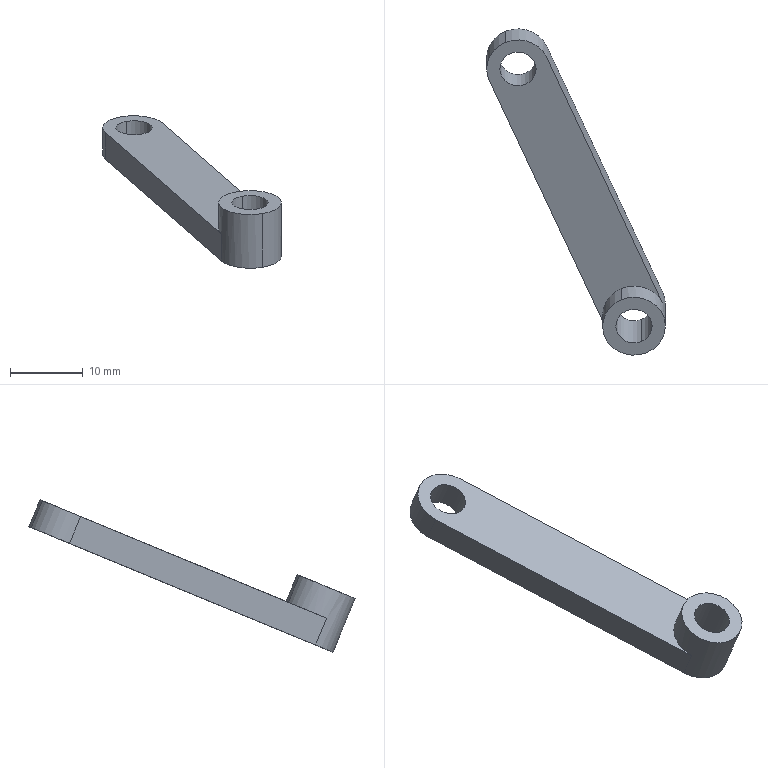Component | SolidWorks | ConnectingRod-B-1 | 1 solid | 13 faces | box 24.62 x 44.93 x 21 mm | volume 1615 mm3 | cylinder 8 | plane 5 | commonest cylinder face diameters 5 x4 8.636 x4
build123d program:
from build123d import *

# Parameters (mm, degrees)
SKETCH1_R           = 2.5
BOSS_EXTRUDE1_DEPTH = 2
SKETCH2_R           = 4.318
SKETCH2_R_2         = 2.5
BOSS_EXTRUDE2_DEPTH = 4


with BuildPart() as part:
    # Sketch1 → Boss-Extrude1 (new, symmetric)
    with BuildSketch(Plane.XY):
        with BuildLine():
            Line((0, 4.318), (40, 4.318))
            ThreePointArc((40, 4.318), (44.318, 0), (40, -4.318))
            Line((40, -4.318), (0, -4.318))
            ThreePointArc((0, -4.318), (-4.318, 0), (0, 4.318))
        make_face()
        Circle(SKETCH1_R, mode=Mode.SUBTRACT)
        with Locations((40, 0)):
            Circle(SKETCH1_R, mode=Mode.SUBTRACT)
    extrude(amount=BOSS_EXTRUDE1_DEPTH, both=True)

    # Sketch2 → Boss-Extrude2 (add)
    with BuildSketch(Plane.XY.offset(2)):
        with Locations(Location((40, 0, 0), (0, 0, 90))):
            Circle(SKETCH2_R)
        with Locations((40, 0)):
            Circle(SKETCH2_R_2, mode=Mode.SUBTRACT)
    extrude(amount=BOSS_EXTRUDE2_DEPTH)


solid = part.part

# Placed as in the assembly
solid = solid.moved(Location((321.124, 13.827, -7.578), (22.448, 0, -66.452)))
STEP:
#1=COLOUR_RGB('',0.7922,0.8196,0.9333);
#2=FILL_AREA_STYLE_COLOUR('',#1);
#3=FILL_AREA_STYLE('',(#2));
#4=SURFACE_STYLE_FILL_AREA(#3);
#5=SURFACE_SIDE_STYLE('',(#4));
#6=SURFACE_STYLE_USAGE(.BOTH.,#5);
#7=PRESENTATION_STYLE_ASSIGNMENT((#6));
#8=CARTESIAN_POINT('',(13.233,-0.7967,-0.5968));
#9=VERTEX_POINT('',#8);
#10=CARTESIAN_POINT('',(13.311,-0.9635,-0.6657));
#11=VERTEX_POINT('',#10);
#12=CARTESIAN_POINT('',(13.272,-0.8801,-0.6313));
#13=DIRECTION('',(0.,-0.3818,0.9242));
#14=DIRECTION('',(0.3995,-0.8473,-0.3501));
#15=AXIS2_PLACEMENT_3D('',#12,#13,#14);
#16=CIRCLE('',#15,0.09843);
#17=EDGE_CURVE('',#9,#11,#16,.T.);
#18=ORIENTED_EDGE('',*,*,#17,.T.);
#19=CARTESIAN_POINT('',(13.311,-0.8432,-0.9568));
#20=VERTEX_POINT('',#19);
#21=CARTESIAN_POINT('',(13.311,-0.9034,-0.8113));
#22=DIRECTION('',(-0.,0.3818,-0.9242));
#23=VECTOR('',#22,39.37);
#24=LINE('',#21,#23);
#25=EDGE_CURVE('',#11,#20,#24,.T.);
#26=ORIENTED_EDGE('',*,*,#25,.T.);
#27=CARTESIAN_POINT('',(13.233,-0.6764,-0.8879));
#28=VERTEX_POINT('',#27);
#29=CARTESIAN_POINT('',(13.272,-0.7598,-0.9224));
#30=DIRECTION('',(0.,-0.3818,0.9242));
#31=DIRECTION('',(0.3995,-0.8473,-0.3501));
#32=AXIS2_PLACEMENT_3D('',#29,#30,#31);
#33=CIRCLE('',#32,0.09843);
#34=EDGE_CURVE('',#28,#20,#33,.T.);
#35=ORIENTED_EDGE('',*,*,#34,.F.);
#36=CARTESIAN_POINT('',(13.233,-0.7366,-0.7424));
#37=DIRECTION('',(-0.,0.3818,-0.9242));
#38=VECTOR('',#37,39.37);
#39=LINE('',#36,#38);
#40=EDGE_CURVE('',#9,#28,#39,.T.);
#41=ORIENTED_EDGE('',*,*,#40,.F.);
#42=EDGE_LOOP('',(#18,#26,#35,#41));
#43=FACE_OUTER_BOUND('',#42,.T.);
#44=CARTESIAN_POINT('',(13.272,-0.82,-0.7768));
#45=DIRECTION('',(-0.,0.3818,-0.9242));
#46=DIRECTION('',(-0.3995,0.8473,0.3501));
#47=AXIS2_PLACEMENT_3D('',#44,#45,#46);
#48=CYLINDRICAL_SURFACE('',#47,0.09843);
#49=ADVANCED_FACE('',(#43),#48,.F.);
#50=CARTESIAN_POINT('',(12.603,0.5977,-0.1911));
#51=VERTEX_POINT('',#50);
#52=CARTESIAN_POINT('',(12.682,0.4309,-0.26));
#53=VERTEX_POINT('',#52);
#54=CARTESIAN_POINT('',(12.643,0.5143,-0.2256));
#55=DIRECTION('',(0.,-0.3818,0.9242));
#56=DIRECTION('',(0.3995,-0.8473,-0.3501));
#57=AXIS2_PLACEMENT_3D('',#54,#55,#56);
#58=CIRCLE('',#57,0.09843);
#59=EDGE_CURVE('',#51,#53,#58,.T.);
#60=ORIENTED_EDGE('',*,*,#59,.T.);
#61=CARTESIAN_POINT('',(12.682,0.491,-0.4056));
#62=VERTEX_POINT('',#61);
#63=CARTESIAN_POINT('',(12.682,0.4309,-0.26));
#64=DIRECTION('',(-0.,0.3818,-0.9242));
#65=VECTOR('',#64,39.37);
#66=LINE('',#63,#65);
#67=EDGE_CURVE('',#53,#62,#66,.T.);
#68=ORIENTED_EDGE('',*,*,#67,.T.);
#69=CARTESIAN_POINT('',(12.603,0.6578,-0.3367));
#70=VERTEX_POINT('',#69);
#71=CARTESIAN_POINT('',(12.643,0.5744,-0.3711));
#72=DIRECTION('',(0.,-0.3818,0.9242));
#73=DIRECTION('',(0.3995,-0.8473,-0.3501));
#74=AXIS2_PLACEMENT_3D('',#71,#72,#73);
#75=CIRCLE('',#74,0.09843);
#76=EDGE_CURVE('',#70,#62,#75,.T.);
#77=ORIENTED_EDGE('',*,*,#76,.F.);
#78=CARTESIAN_POINT('',(12.603,0.5977,-0.1911));
#79=DIRECTION('',(-0.,0.3818,-0.9242));
#80=VECTOR('',#79,39.37);
#81=LINE('',#78,#80);
#82=EDGE_CURVE('',#51,#70,#81,.T.);
#83=ORIENTED_EDGE('',*,*,#82,.F.);
#84=EDGE_LOOP('',(#60,#68,#77,#83));
#85=FACE_OUTER_BOUND('',#84,.T.);
#86=CARTESIAN_POINT('',(12.643,0.5143,-0.2256));
#87=DIRECTION('',(-0.,0.3818,-0.9242));
#88=DIRECTION('',(-0.3995,0.8473,0.3501));
#89=AXIS2_PLACEMENT_3D('',#86,#87,#88);
#90=CYLINDRICAL_SURFACE('',#89,0.09843);
#91=ADVANCED_FACE('',(#85),#90,.F.);
#92=CARTESIAN_POINT('',(13.34,-1.024,-0.6908));
#93=VERTEX_POINT('',#92);
#94=CARTESIAN_POINT('',(13.204,-0.7361,-0.5718));
#95=VERTEX_POINT('',#94);
#96=CARTESIAN_POINT('',(13.272,-0.8801,-0.6313));
#97=DIRECTION('',(0.,-0.3818,0.9242));
#98=DIRECTION('',(0.3995,-0.8473,-0.3501));
#99=AXIS2_PLACEMENT_3D('',#96,#97,#98);
#100=CIRCLE('',#99,0.17);
#101=EDGE_CURVE('',#93,#95,#100,.T.);
#102=ORIENTED_EDGE('',*,*,#101,.F.);
#103=CARTESIAN_POINT('',(13.34,-0.9039,-0.9819));
#104=VERTEX_POINT('',#103);
#105=CARTESIAN_POINT('',(13.34,-0.964,-0.8363));
#106=DIRECTION('',(-0.,0.3818,-0.9242));
#107=VECTOR('',#106,39.37);
#108=LINE('',#105,#107);
#109=EDGE_CURVE('',#93,#104,#108,.T.);
#110=ORIENTED_EDGE('',*,*,#109,.T.);
#111=CARTESIAN_POINT('',(13.428,-0.6971,-0.8964));
#112=VERTEX_POINT('',#111);
#113=CARTESIAN_POINT('',(13.272,-0.7598,-0.9224));
#114=DIRECTION('',(0.,-0.3818,0.9242));
#115=DIRECTION('',(0.3995,-0.8473,-0.3501));
#116=AXIS2_PLACEMENT_3D('',#113,#114,#115);
#117=CIRCLE('',#116,0.17);
#118=EDGE_CURVE('',#104,#112,#117,.T.);
#119=ORIENTED_EDGE('',*,*,#118,.T.);
#120=CARTESIAN_POINT('',(13.428,-0.7572,-0.7509));
#121=VERTEX_POINT('',#120);
#122=CARTESIAN_POINT('',(13.428,-0.7572,-0.7509));
#123=DIRECTION('',(-0.,0.3818,-0.9242));
#124=VECTOR('',#123,39.37);
#125=LINE('',#122,#124);
#126=EDGE_CURVE('',#121,#112,#125,.T.);
#127=ORIENTED_EDGE('',*,*,#126,.F.);
#128=CARTESIAN_POINT('',(13.204,-0.6759,-0.7173));
#129=VERTEX_POINT('',#128);
#130=CARTESIAN_POINT('',(13.272,-0.82,-0.7768));
#131=DIRECTION('',(0.,-0.3818,0.9242));
#132=DIRECTION('',(0.3995,-0.8473,-0.3501));
#133=AXIS2_PLACEMENT_3D('',#130,#131,#132);
#134=CIRCLE('',#133,0.17);
#135=EDGE_CURVE('',#121,#129,#134,.T.);
#136=ORIENTED_EDGE('',*,*,#135,.T.);
#137=CARTESIAN_POINT('',(13.204,-0.6759,-0.7173));
#138=DIRECTION('',(-0.,0.3818,-0.9242));
#139=VECTOR('',#138,39.37);
#140=LINE('',#137,#139);
#141=EDGE_CURVE('',#95,#129,#140,.T.);
#142=ORIENTED_EDGE('',*,*,#141,.F.);
#143=EDGE_LOOP('',(#102,#110,#119,#127,#136,#142));
#144=FACE_OUTER_BOUND('',#143,.T.);
#145=CARTESIAN_POINT('',(13.272,-0.82,-0.7768));
#146=DIRECTION('',(-0.,0.3818,-0.9242));
#147=DIRECTION('',(-0.3995,0.8473,0.3501));
#148=AXIS2_PLACEMENT_3D('',#145,#146,#147);
#149=CYLINDRICAL_SURFACE('',#148,0.17);
#150=ADVANCED_FACE('',(#144),#149,.T.);
#151=CARTESIAN_POINT('',(12.575,0.6583,-0.1661));
#152=VERTEX_POINT('',#151);
#153=CARTESIAN_POINT('',(12.487,0.4515,-0.2515));
#154=VERTEX_POINT('',#153);
#155=CARTESIAN_POINT('',(12.643,0.5143,-0.2256));
#156=DIRECTION('',(0.,-0.3818,0.9242));
#157=DIRECTION('',(0.3995,-0.8473,-0.3501));
#158=AXIS2_PLACEMENT_3D('',#155,#156,#157);
#159=CIRCLE('',#158,0.17);
#160=EDGE_CURVE('',#152,#154,#159,.T.);
#161=ORIENTED_EDGE('',*,*,#160,.F.);
#162=CARTESIAN_POINT('',(12.575,0.7185,-0.3116));
#163=VERTEX_POINT('',#162);
#164=CARTESIAN_POINT('',(12.575,0.6583,-0.1661));
#165=DIRECTION('',(-0.,0.3818,-0.9242));
#166=VECTOR('',#165,39.37);
#167=LINE('',#164,#166);
#168=EDGE_CURVE('',#152,#163,#167,.T.);
#169=ORIENTED_EDGE('',*,*,#168,.T.);
#170=CARTESIAN_POINT('',(12.487,0.5117,-0.397));
#171=VERTEX_POINT('',#170);
#172=CARTESIAN_POINT('',(12.643,0.5744,-0.3711));
#173=DIRECTION('',(0.,-0.3818,0.9242));
#174=DIRECTION('',(0.3995,-0.8473,-0.3501));
#175=AXIS2_PLACEMENT_3D('',#172,#173,#174);
#176=CIRCLE('',#175,0.17);
#177=EDGE_CURVE('',#163,#171,#176,.T.);
#178=ORIENTED_EDGE('',*,*,#177,.T.);
#179=CARTESIAN_POINT('',(12.487,0.4515,-0.2515));
#180=DIRECTION('',(-0.,0.3818,-0.9242));
#181=VECTOR('',#180,39.37);
#182=LINE('',#179,#181);
#183=EDGE_CURVE('',#154,#171,#182,.T.);
#184=ORIENTED_EDGE('',*,*,#183,.F.);
#185=EDGE_LOOP('',(#161,#169,#178,#184));
#186=FACE_OUTER_BOUND('',#185,.T.);
#187=CARTESIAN_POINT('',(12.643,0.5143,-0.2256));
#188=DIRECTION('',(-0.,0.3818,-0.9242));
#189=DIRECTION('',(-0.3995,0.8473,0.3501));
#190=AXIS2_PLACEMENT_3D('',#187,#188,#189);
#191=CYLINDRICAL_SURFACE('',#190,0.17);
#192=ADVANCED_FACE('',(#186),#191,.T.);
#193=ORIENTED_EDGE('',*,*,#135,.F.);
#194=CARTESIAN_POINT('',(12.799,0.5771,-0.1996));
#195=VERTEX_POINT('',#194);
#196=CARTESIAN_POINT('',(12.799,0.5771,-0.1996));
#197=DIRECTION('',(-0.3995,0.8473,0.3501));
#198=VECTOR('',#197,39.37);
#199=LINE('',#196,#198);
#200=EDGE_CURVE('',#121,#195,#199,.T.);
#201=ORIENTED_EDGE('',*,*,#200,.T.);
#202=CARTESIAN_POINT('',(12.643,0.5143,-0.2256));
#203=DIRECTION('',(0.,-0.3818,0.9242));
#204=DIRECTION('',(0.3995,-0.8473,-0.3501));
#205=AXIS2_PLACEMENT_3D('',#202,#203,#204);
#206=CIRCLE('',#205,0.17);
#207=EDGE_CURVE('',#195,#152,#206,.T.);
#208=ORIENTED_EDGE('',*,*,#207,.T.);
#209=ORIENTED_EDGE('',*,*,#160,.T.);
#210=CARTESIAN_POINT('',(13.116,-0.8827,-0.8028));
#211=VERTEX_POINT('',#210);
#212=CARTESIAN_POINT('',(12.487,0.4515,-0.2515));
#213=DIRECTION('',(0.3995,-0.8473,-0.3501));
#214=VECTOR('',#213,39.37);
#215=LINE('',#212,#214);
#216=EDGE_CURVE('',#154,#211,#215,.T.);
#217=ORIENTED_EDGE('',*,*,#216,.T.);
#218=CARTESIAN_POINT('',(13.272,-0.82,-0.7768));
#219=DIRECTION('',(0.,-0.3818,0.9242));
#220=DIRECTION('',(0.3995,-0.8473,-0.3501));
#221=AXIS2_PLACEMENT_3D('',#218,#219,#220);
#222=CIRCLE('',#221,0.17);
#223=EDGE_CURVE('',#129,#211,#222,.T.);
#224=ORIENTED_EDGE('',*,*,#223,.F.);
#225=EDGE_LOOP('',(#193,#201,#208,#209,#217,#224));
#226=FACE_OUTER_BOUND('',#225,.T.);
#227=ORIENTED_EDGE('',*,*,#59,.F.);
#228=CARTESIAN_POINT('',(12.643,0.5143,-0.2256));
#229=DIRECTION('',(0.,-0.3818,0.9242));
#230=DIRECTION('',(0.3995,-0.8473,-0.3501));
#231=AXIS2_PLACEMENT_3D('',#228,#229,#230);
#232=CIRCLE('',#231,0.09843);
#233=EDGE_CURVE('',#53,#51,#232,.T.);
#234=ORIENTED_EDGE('',*,*,#233,.F.);
#235=EDGE_LOOP('',(#227,#234));
#236=FACE_BOUND('',#235,.T.);
#237=CARTESIAN_POINT('',(12.643,0.5143,-0.2256));
#238=DIRECTION('',(0.,-0.3818,0.9242));
#239=DIRECTION('',(0.3995,-0.8473,-0.3501));
#240=AXIS2_PLACEMENT_3D('',#237,#238,#239);
#241=PLANE('',#240);
#242=ADVANCED_FACE('',(#226,#236),#241,.T.);
#243=CARTESIAN_POINT('',(12.799,0.6372,-0.3452));
#244=VERTEX_POINT('',#243);
#245=CARTESIAN_POINT('',(12.643,0.5744,-0.3711));
#246=DIRECTION('',(0.,-0.3818,0.9242));
#247=DIRECTION('',(0.3995,-0.8473,-0.3501));
#248=AXIS2_PLACEMENT_3D('',#245,#246,#247);
#249=CIRCLE('',#248,0.17);
#250=EDGE_CURVE('',#244,#163,#249,.T.);
#251=ORIENTED_EDGE('',*,*,#250,.F.);
#252=CARTESIAN_POINT('',(12.799,0.6372,-0.3452));
#253=DIRECTION('',(-0.3995,0.8473,0.3501));
#254=VECTOR('',#253,39.37);
#255=LINE('',#252,#254);
#256=EDGE_CURVE('',#112,#244,#255,.T.);
#257=ORIENTED_EDGE('',*,*,#256,.F.);
#258=ORIENTED_EDGE('',*,*,#118,.F.);
#259=CARTESIAN_POINT('',(13.116,-0.8226,-0.9483));
#260=VERTEX_POINT('',#259);
#261=CARTESIAN_POINT('',(13.272,-0.7598,-0.9224));
#262=DIRECTION('',(0.,-0.3818,0.9242));
#263=DIRECTION('',(0.3995,-0.8473,-0.3501));
#264=AXIS2_PLACEMENT_3D('',#261,#262,#263);
#265=CIRCLE('',#264,0.17);
#266=EDGE_CURVE('',#260,#104,#265,.T.);
#267=ORIENTED_EDGE('',*,*,#266,.F.);
#268=CARTESIAN_POINT('',(12.487,0.5117,-0.397));
#269=DIRECTION('',(0.3995,-0.8473,-0.3501));
#270=VECTOR('',#269,39.37);
#271=LINE('',#268,#270);
#272=EDGE_CURVE('',#171,#260,#271,.T.);
#273=ORIENTED_EDGE('',*,*,#272,.F.);
#274=ORIENTED_EDGE('',*,*,#177,.F.);
#275=EDGE_LOOP('',(#251,#257,#258,#267,#273,#274));
#276=FACE_OUTER_BOUND('',#275,.T.);
#277=ORIENTED_EDGE('',*,*,#76,.T.);
#278=CARTESIAN_POINT('',(12.643,0.5744,-0.3711));
#279=DIRECTION('',(0.,-0.3818,0.9242));
#280=DIRECTION('',(0.3995,-0.8473,-0.3501));
#281=AXIS2_PLACEMENT_3D('',#278,#279,#280);
#282=CIRCLE('',#281,0.09843);
#283=EDGE_CURVE('',#62,#70,#282,.T.);
#284=ORIENTED_EDGE('',*,*,#283,.T.);
#285=EDGE_LOOP('',(#277,#284));
#286=FACE_BOUND('',#285,.T.);
#287=ORIENTED_EDGE('',*,*,#34,.T.);
#288=CARTESIAN_POINT('',(13.272,-0.7598,-0.9224));
#289=DIRECTION('',(0.,-0.3818,0.9242));
#290=DIRECTION('',(0.3995,-0.8473,-0.3501));
#291=AXIS2_PLACEMENT_3D('',#288,#289,#290);
#292=CIRCLE('',#291,0.09843);
#293=EDGE_CURVE('',#20,#28,#292,.T.);
#294=ORIENTED_EDGE('',*,*,#293,.T.);
#295=EDGE_LOOP('',(#287,#294));
#296=FACE_BOUND('',#295,.T.);
#297=CARTESIAN_POINT('',(12.643,0.5744,-0.3711));
#298=DIRECTION('',(0.,-0.3818,0.9242));
#299=DIRECTION('',(0.3995,-0.8473,-0.3501));
#300=AXIS2_PLACEMENT_3D('',#297,#298,#299);
#301=PLANE('',#300);
#302=ADVANCED_FACE('',(#276,#286,#296),#301,.F.);
#303=ORIENTED_EDGE('',*,*,#168,.F.);
#304=ORIENTED_EDGE('',*,*,#207,.F.);
#305=CARTESIAN_POINT('',(12.799,0.5771,-0.1996));
#306=DIRECTION('',(-0.,0.3818,-0.9242));
#307=VECTOR('',#306,39.37);
#308=LINE('',#305,#307);
#309=EDGE_CURVE('',#195,#244,#308,.T.);
#310=ORIENTED_EDGE('',*,*,#309,.T.);
#311=ORIENTED_EDGE('',*,*,#250,.T.);
#312=EDGE_LOOP('',(#303,#304,#310,#311));
#313=FACE_OUTER_BOUND('',#312,.T.);
#314=CARTESIAN_POINT('',(12.643,0.5143,-0.2256));
#315=DIRECTION('',(-0.,0.3818,-0.9242));
#316=DIRECTION('',(-0.3995,0.8473,0.3501));
#317=AXIS2_PLACEMENT_3D('',#314,#315,#316);
#318=CYLINDRICAL_SURFACE('',#317,0.17);
#319=ADVANCED_FACE('',(#313),#318,.T.);
#320=ORIENTED_EDGE('',*,*,#272,.T.);
#321=CARTESIAN_POINT('',(13.116,-0.8827,-0.8028));
#322=DIRECTION('',(-0.,0.3818,-0.9242));
#323=VECTOR('',#322,39.37);
#324=LINE('',#321,#323);
#325=EDGE_CURVE('',#211,#260,#324,.T.);
#326=ORIENTED_EDGE('',*,*,#325,.F.);
#327=ORIENTED_EDGE('',*,*,#216,.F.);
#328=ORIENTED_EDGE('',*,*,#183,.T.);
#329=EDGE_LOOP('',(#320,#326,#327,#328));
#330=FACE_OUTER_BOUND('',#329,.T.);
#331=CARTESIAN_POINT('',(12.487,0.4515,-0.2515));
#332=DIRECTION('',(0.9167,0.3692,0.1526));
#333=DIRECTION('',(0.,-0.3818,0.9242));
#334=AXIS2_PLACEMENT_3D('',#331,#332,#333);
#335=PLANE('',#334);
#336=ADVANCED_FACE('',(#330),#335,.F.);
#337=ORIENTED_EDGE('',*,*,#109,.F.);
#338=CARTESIAN_POINT('',(13.272,-0.8801,-0.6313));
#339=DIRECTION('',(0.,-0.3818,0.9242));
#340=DIRECTION('',(0.3995,-0.8473,-0.3501));
#341=AXIS2_PLACEMENT_3D('',#338,#339,#340);
#342=CIRCLE('',#341,0.17);
#343=EDGE_CURVE('',#95,#93,#342,.T.);
#344=ORIENTED_EDGE('',*,*,#343,.F.);
#345=ORIENTED_EDGE('',*,*,#141,.T.);
#346=ORIENTED_EDGE('',*,*,#223,.T.);
#347=ORIENTED_EDGE('',*,*,#325,.T.);
#348=ORIENTED_EDGE('',*,*,#266,.T.);
#349=EDGE_LOOP('',(#337,#344,#345,#346,#347,#348));
#350=FACE_OUTER_BOUND('',#349,.T.);
#351=CARTESIAN_POINT('',(13.272,-0.82,-0.7768));
#352=DIRECTION('',(-0.,0.3818,-0.9242));
#353=DIRECTION('',(-0.3995,0.8473,0.3501));
#354=AXIS2_PLACEMENT_3D('',#351,#352,#353);
#355=CYLINDRICAL_SURFACE('',#354,0.17);
#356=ADVANCED_FACE('',(#350),#355,.T.);
#357=ORIENTED_EDGE('',*,*,#256,.T.);
#358=ORIENTED_EDGE('',*,*,#309,.F.);
#359=ORIENTED_EDGE('',*,*,#200,.F.);
#360=ORIENTED_EDGE('',*,*,#126,.T.);
#361=EDGE_LOOP('',(#357,#358,#359,#360));
#362=FACE_OUTER_BOUND('',#361,.T.);
#363=CARTESIAN_POINT('',(12.799,0.5771,-0.1996));
#364=DIRECTION('',(-0.9167,-0.3692,-0.1526));
#365=DIRECTION('',(-0.,0.3818,-0.9242));
#366=AXIS2_PLACEMENT_3D('',#363,#364,#365);
#367=PLANE('',#366);
#368=ADVANCED_FACE('',(#362),#367,.F.);
#369=ORIENTED_EDGE('',*,*,#67,.F.);
#370=ORIENTED_EDGE('',*,*,#233,.T.);
#371=ORIENTED_EDGE('',*,*,#82,.T.);
#372=ORIENTED_EDGE('',*,*,#283,.F.);
#373=EDGE_LOOP('',(#369,#370,#371,#372));
#374=FACE_OUTER_BOUND('',#373,.T.);
#375=CARTESIAN_POINT('',(12.643,0.5143,-0.2256));
#376=DIRECTION('',(-0.,0.3818,-0.9242));
#377=DIRECTION('',(-0.3995,0.8473,0.3501));
#378=AXIS2_PLACEMENT_3D('',#375,#376,#377);
#379=CYLINDRICAL_SURFACE('',#378,0.09843);
#380=ADVANCED_FACE('',(#374),#379,.F.);
#381=ORIENTED_EDGE('',*,*,#25,.F.);
#382=CARTESIAN_POINT('',(13.272,-0.8801,-0.6313));
#383=DIRECTION('',(0.,-0.3818,0.9242));
#384=DIRECTION('',(0.3995,-0.8473,-0.3501));
#385=AXIS2_PLACEMENT_3D('',#382,#383,#384);
#386=CIRCLE('',#385,0.09843);
#387=EDGE_CURVE('',#11,#9,#386,.T.);
#388=ORIENTED_EDGE('',*,*,#387,.T.);
#389=ORIENTED_EDGE('',*,*,#40,.T.);
#390=ORIENTED_EDGE('',*,*,#293,.F.);
#391=EDGE_LOOP('',(#381,#388,#389,#390));
#392=FACE_OUTER_BOUND('',#391,.T.);
#393=CARTESIAN_POINT('',(13.272,-0.82,-0.7768));
#394=DIRECTION('',(-0.,0.3818,-0.9242));
#395=DIRECTION('',(-0.3995,0.8473,0.3501));
#396=AXIS2_PLACEMENT_3D('',#393,#394,#395);
#397=CYLINDRICAL_SURFACE('',#396,0.09843);
#398=ADVANCED_FACE('',(#392),#397,.F.);
#399=ORIENTED_EDGE('',*,*,#343,.T.);
#400=ORIENTED_EDGE('',*,*,#101,.T.);
#401=EDGE_LOOP('',(#399,#400));
#402=FACE_OUTER_BOUND('',#401,.T.);
#403=ORIENTED_EDGE('',*,*,#17,.F.);
#404=ORIENTED_EDGE('',*,*,#387,.F.);
#405=EDGE_LOOP('',(#403,#404));
#406=FACE_BOUND('',#405,.T.);
#407=CARTESIAN_POINT('',(13.272,-0.8801,-0.6313));
#408=DIRECTION('',(0.,-0.3818,0.9242));
#409=DIRECTION('',(0.3995,-0.8473,-0.3501));
#410=AXIS2_PLACEMENT_3D('',#407,#408,#409);
#411=PLANE('',#410);
#412=ADVANCED_FACE('',(#402,#406),#411,.T.);
#413=CLOSED_SHELL('',(#49,#91,#150,#192,#242,#302,#319,#336,#356,#368,#380,#398,#412));
#414=MANIFOLD_SOLID_BREP('',#413);
#415=STYLED_ITEM('',(#7),#414);
#416=PRESENTATION_LAYER_ASSIGNMENT('','',(#415));
#417=CARTESIAN_POINT('',(0.,0.,0.));
#418=DIRECTION('',(0.,0.,1.));
#419=DIRECTION('',(1.,0.,0.));
#420=AXIS2_PLACEMENT_3D('',#417,#418,#419);
#421=(LENGTH_UNIT()NAMED_UNIT(*)SI_UNIT($,.METRE.));
#422=LENGTH_MEASURE_WITH_UNIT(LENGTH_MEASURE(0.0254),#421);
#423=DIMENSIONAL_EXPONENTS(1.,0.,0.,0.,0.,0.,0.);
#424=(CONVERSION_BASED_UNIT('',#422)LENGTH_UNIT()NAMED_UNIT(#423));
#425=UNCERTAINTY_MEASURE_WITH_UNIT(LENGTH_MEASURE(0.00001),#424,'','');
#426=(NAMED_UNIT(*)PLANE_ANGLE_UNIT()SI_UNIT($,.RADIAN.));
#427=(NAMED_UNIT(*)SI_UNIT($,.STERADIAN.)SOLID_ANGLE_UNIT());
#428=(GEOMETRIC_REPRESENTATION_CONTEXT(3)GLOBAL_UNCERTAINTY_ASSIGNED_CONTEXT((#425))GLOBAL_UNIT_ASSIGNED_CONTEXT((#424,#426,#427))REPRESENTATION_CONTEXT('',''));
#429=ADVANCED_BREP_SHAPE_REPRESENTATION('',(#414,#420),#428);
#430=(LENGTH_UNIT()NAMED_UNIT(*)SI_UNIT($,.METRE.));
#431=LENGTH_MEASURE_WITH_UNIT(LENGTH_MEASURE(0.0254),#430);
#432=DIMENSIONAL_EXPONENTS(1.,0.,0.,0.,0.,0.,0.);
#433=(CONVERSION_BASED_UNIT('',#431)LENGTH_UNIT()NAMED_UNIT(#432));
#434=UNCERTAINTY_MEASURE_WITH_UNIT(LENGTH_MEASURE(0.00001),#433,'','');
#435=(NAMED_UNIT(*)PLANE_ANGLE_UNIT()SI_UNIT($,.RADIAN.));
#436=(NAMED_UNIT(*)SI_UNIT($,.STERADIAN.)SOLID_ANGLE_UNIT());
#437=(GEOMETRIC_REPRESENTATION_CONTEXT(3)GLOBAL_UNCERTAINTY_ASSIGNED_CONTEXT((#434))GLOBAL_UNIT_ASSIGNED_CONTEXT((#433,#435,#436))REPRESENTATION_CONTEXT('',''));
#438=MECHANICAL_DESIGN_GEOMETRIC_PRESENTATION_REPRESENTATION('',(#415),#437);